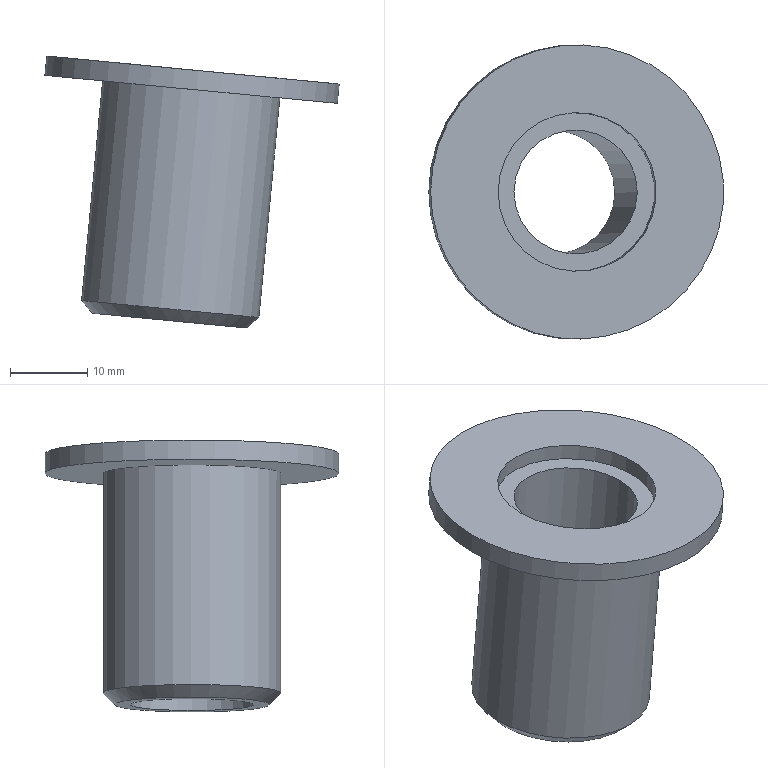Component | NX | DINGTAO | 1 solid | 9 faces | volume 8429 mm3 | plane 4 | cylinder 4 | cone 1 | commonest cylinder face diameters 38 x1 23 x1 16 x1 20.5 x1